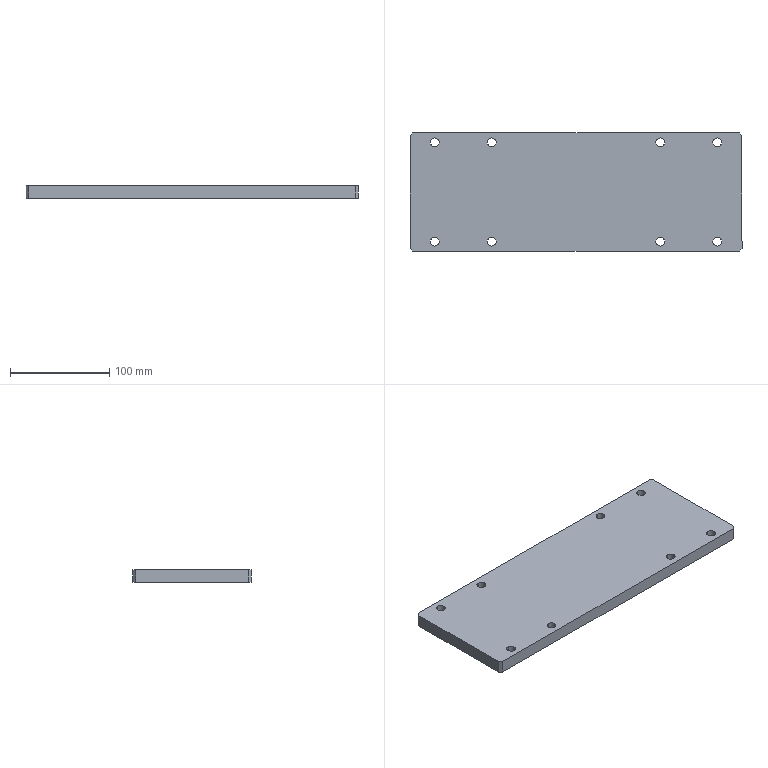Component | SolidWorks | STE21014.01-42-2 | 1 solid | 26 faces | box 335 x 120 x 13 mm | volume 515750 mm3 | cylinder 16 | plane 10 | commonest cylinder face diameters 9 x16 | material Q235
build123d program:
from build123d import *

# Parameters (mm, degrees)
SKETCH1_W            = 335
SKETCH1_H            = 120
BOSS_EXTRUDE1_DEPTH  = 13
M8_CLEARANCE_HOLE1_D = 9
CHAMFER1_SIZE        = 3


with BuildPart() as part:
    # Sketch1 → Boss-Extrude1 (new body)
    with BuildSketch(Plane(origin=(0, 0, 0), x_dir=(1, 0, 0), z_dir=(0, 1, 0))):
        Rectangle(SKETCH1_W, SKETCH1_H)
    extrude(amount=BOSS_EXTRUDE1_DEPTH)

    # M8 Clearance Hole1 (through all)
    with Locations(Plane(origin=(0, 13, 0), x_dir=(1, 0, 0), z_dir=(0, 1, 0))):
        with Locations((-142.5, -50), (-85, -50), (85, -50), (142.5, -50), (-142.5, 50), (-85, 50), (85, 50), (142.5, 50)):
            Hole(M8_CLEARANCE_HOLE1_D / 2)

    # Chamfer1
    chamfer1_edges = [part.edges().sort_by_distance(p)[0] for p in [
        (-167.5, 6.5, -60),
        (167.5, 6.5, -60),
        (167.5, 6.5, 60),
        (-167.5, 6.5, 60),
    ]]
    chamfer(chamfer1_edges, length=CHAMFER1_SIZE)


solid = part.part

# Placed as in the assembly
solid = solid.moved(Location((137.5, 890, -673), (90, 0, 0)))
STEP:
#1=COLOUR_RGB('',0.7922,0.8196,0.9333);
#2=FILL_AREA_STYLE_COLOUR('',#1);
#3=FILL_AREA_STYLE('',(#2));
#4=SURFACE_STYLE_FILL_AREA(#3);
#5=SURFACE_SIDE_STYLE('',(#4));
#6=SURFACE_STYLE_USAGE(.BOTH.,#5);
#7=PRESENTATION_STYLE_ASSIGNMENT((#6));
#8=CARTESIAN_POINT('',(-0.1969,36.831,-25.984));
#9=VERTEX_POINT('',#8);
#10=CARTESIAN_POINT('',(-0.1969,37.185,-25.984));
#11=VERTEX_POINT('',#10);
#12=CARTESIAN_POINT('',(-0.1969,37.008,-25.984));
#13=DIRECTION('',(0.,-0.,-1.));
#14=DIRECTION('',(-0.,1.,0.));
#15=AXIS2_PLACEMENT_3D('',#12,#13,#14);
#16=CIRCLE('',#15,0.1772);
#17=EDGE_CURVE('',#9,#11,#16,.T.);
#18=ORIENTED_EDGE('',*,*,#17,.F.);
#19=CARTESIAN_POINT('',(-0.1969,36.831,-26.496));
#20=VERTEX_POINT('',#19);
#21=CARTESIAN_POINT('',(-0.1969,36.831,-26.496));
#22=DIRECTION('',(0.,-0.,-1.));
#23=VECTOR('',#22,39.37);
#24=LINE('',#21,#23);
#25=EDGE_CURVE('',#9,#20,#24,.T.);
#26=ORIENTED_EDGE('',*,*,#25,.T.);
#27=CARTESIAN_POINT('',(-0.1969,37.185,-26.496));
#28=VERTEX_POINT('',#27);
#29=CARTESIAN_POINT('',(-0.1969,37.008,-26.496));
#30=DIRECTION('',(0.,-0.,-1.));
#31=DIRECTION('',(-0.,1.,0.));
#32=AXIS2_PLACEMENT_3D('',#29,#30,#31);
#33=CIRCLE('',#32,0.1772);
#34=EDGE_CURVE('',#20,#28,#33,.T.);
#35=ORIENTED_EDGE('',*,*,#34,.T.);
#36=CARTESIAN_POINT('',(-0.1969,37.185,-26.496));
#37=DIRECTION('',(0.,-0.,-1.));
#38=VECTOR('',#37,39.37);
#39=LINE('',#36,#38);
#40=EDGE_CURVE('',#11,#28,#39,.T.);
#41=ORIENTED_EDGE('',*,*,#40,.F.);
#42=EDGE_LOOP('',(#18,#26,#35,#41));
#43=FACE_OUTER_BOUND('',#42,.T.);
#44=CARTESIAN_POINT('',(-0.1969,37.008,-26.496));
#45=DIRECTION('',(0.,-0.,-1.));
#46=DIRECTION('',(-0.,1.,0.));
#47=AXIS2_PLACEMENT_3D('',#44,#45,#46);
#48=CYLINDRICAL_SURFACE('',#47,0.1772);
#49=ADVANCED_FACE('',(#43),#48,.F.);
#50=CARTESIAN_POINT('',(2.067,36.831,-25.984));
#51=VERTEX_POINT('',#50);
#52=CARTESIAN_POINT('',(2.067,37.185,-25.984));
#53=VERTEX_POINT('',#52);
#54=CARTESIAN_POINT('',(2.067,37.008,-25.984));
#55=DIRECTION('',(0.,-0.,-1.));
#56=DIRECTION('',(-0.,1.,0.));
#57=AXIS2_PLACEMENT_3D('',#54,#55,#56);
#58=CIRCLE('',#57,0.1772);
#59=EDGE_CURVE('',#51,#53,#58,.T.);
#60=ORIENTED_EDGE('',*,*,#59,.F.);
#61=CARTESIAN_POINT('',(2.067,36.831,-26.496));
#62=VERTEX_POINT('',#61);
#63=CARTESIAN_POINT('',(2.067,36.831,-26.496));
#64=DIRECTION('',(0.,-0.,-1.));
#65=VECTOR('',#64,39.37);
#66=LINE('',#63,#65);
#67=EDGE_CURVE('',#51,#62,#66,.T.);
#68=ORIENTED_EDGE('',*,*,#67,.T.);
#69=CARTESIAN_POINT('',(2.067,37.185,-26.496));
#70=VERTEX_POINT('',#69);
#71=CARTESIAN_POINT('',(2.067,37.008,-26.496));
#72=DIRECTION('',(0.,-0.,-1.));
#73=DIRECTION('',(-0.,1.,0.));
#74=AXIS2_PLACEMENT_3D('',#71,#72,#73);
#75=CIRCLE('',#74,0.1772);
#76=EDGE_CURVE('',#62,#70,#75,.T.);
#77=ORIENTED_EDGE('',*,*,#76,.T.);
#78=CARTESIAN_POINT('',(2.067,37.185,-26.496));
#79=DIRECTION('',(0.,-0.,-1.));
#80=VECTOR('',#79,39.37);
#81=LINE('',#78,#80);
#82=EDGE_CURVE('',#53,#70,#81,.T.);
#83=ORIENTED_EDGE('',*,*,#82,.F.);
#84=EDGE_LOOP('',(#60,#68,#77,#83));
#85=FACE_OUTER_BOUND('',#84,.T.);
#86=CARTESIAN_POINT('',(2.067,37.008,-26.496));
#87=DIRECTION('',(0.,-0.,-1.));
#88=DIRECTION('',(-0.,1.,0.));
#89=AXIS2_PLACEMENT_3D('',#86,#87,#88);
#90=CYLINDRICAL_SURFACE('',#89,0.1772);
#91=ADVANCED_FACE('',(#85),#90,.F.);
#92=CARTESIAN_POINT('',(8.76,36.831,-25.984));
#93=VERTEX_POINT('',#92);
#94=CARTESIAN_POINT('',(8.76,37.185,-25.984));
#95=VERTEX_POINT('',#94);
#96=CARTESIAN_POINT('',(8.76,37.008,-25.984));
#97=DIRECTION('',(0.,-0.,-1.));
#98=DIRECTION('',(-0.,1.,0.));
#99=AXIS2_PLACEMENT_3D('',#96,#97,#98);
#100=CIRCLE('',#99,0.1772);
#101=EDGE_CURVE('',#93,#95,#100,.T.);
#102=ORIENTED_EDGE('',*,*,#101,.F.);
#103=CARTESIAN_POINT('',(8.76,36.831,-26.496));
#104=VERTEX_POINT('',#103);
#105=CARTESIAN_POINT('',(8.76,36.831,-26.496));
#106=DIRECTION('',(0.,-0.,-1.));
#107=VECTOR('',#106,39.37);
#108=LINE('',#105,#107);
#109=EDGE_CURVE('',#93,#104,#108,.T.);
#110=ORIENTED_EDGE('',*,*,#109,.T.);
#111=CARTESIAN_POINT('',(8.76,37.185,-26.496));
#112=VERTEX_POINT('',#111);
#113=CARTESIAN_POINT('',(8.76,37.008,-26.496));
#114=DIRECTION('',(0.,-0.,-1.));
#115=DIRECTION('',(-0.,1.,0.));
#116=AXIS2_PLACEMENT_3D('',#113,#114,#115);
#117=CIRCLE('',#116,0.1772);
#118=EDGE_CURVE('',#104,#112,#117,.T.);
#119=ORIENTED_EDGE('',*,*,#118,.T.);
#120=CARTESIAN_POINT('',(8.76,37.185,-26.496));
#121=DIRECTION('',(0.,-0.,-1.));
#122=VECTOR('',#121,39.37);
#123=LINE('',#120,#122);
#124=EDGE_CURVE('',#95,#112,#123,.T.);
#125=ORIENTED_EDGE('',*,*,#124,.F.);
#126=EDGE_LOOP('',(#102,#110,#119,#125));
#127=FACE_OUTER_BOUND('',#126,.T.);
#128=CARTESIAN_POINT('',(8.76,37.008,-26.496));
#129=DIRECTION('',(0.,-0.,-1.));
#130=DIRECTION('',(-0.,1.,0.));
#131=AXIS2_PLACEMENT_3D('',#128,#129,#130);
#132=CYLINDRICAL_SURFACE('',#131,0.1772);
#133=ADVANCED_FACE('',(#127),#132,.F.);
#134=CARTESIAN_POINT('',(11.024,36.831,-25.984));
#135=VERTEX_POINT('',#134);
#136=CARTESIAN_POINT('',(11.024,37.185,-25.984));
#137=VERTEX_POINT('',#136);
#138=CARTESIAN_POINT('',(11.024,37.008,-25.984));
#139=DIRECTION('',(0.,-0.,-1.));
#140=DIRECTION('',(0.,1.,0.));
#141=AXIS2_PLACEMENT_3D('',#138,#139,#140);
#142=CIRCLE('',#141,0.1772);
#143=EDGE_CURVE('',#135,#137,#142,.T.);
#144=ORIENTED_EDGE('',*,*,#143,.F.);
#145=CARTESIAN_POINT('',(11.024,36.831,-26.496));
#146=VERTEX_POINT('',#145);
#147=CARTESIAN_POINT('',(11.024,36.831,-26.496));
#148=DIRECTION('',(0.,-0.,-1.));
#149=VECTOR('',#148,39.37);
#150=LINE('',#147,#149);
#151=EDGE_CURVE('',#135,#146,#150,.T.);
#152=ORIENTED_EDGE('',*,*,#151,.T.);
#153=CARTESIAN_POINT('',(11.024,37.185,-26.496));
#154=VERTEX_POINT('',#153);
#155=CARTESIAN_POINT('',(11.024,37.008,-26.496));
#156=DIRECTION('',(0.,-0.,-1.));
#157=DIRECTION('',(0.,1.,0.));
#158=AXIS2_PLACEMENT_3D('',#155,#156,#157);
#159=CIRCLE('',#158,0.1772);
#160=EDGE_CURVE('',#146,#154,#159,.T.);
#161=ORIENTED_EDGE('',*,*,#160,.T.);
#162=CARTESIAN_POINT('',(11.024,37.185,-26.496));
#163=DIRECTION('',(0.,-0.,-1.));
#164=VECTOR('',#163,39.37);
#165=LINE('',#162,#164);
#166=EDGE_CURVE('',#137,#154,#165,.T.);
#167=ORIENTED_EDGE('',*,*,#166,.F.);
#168=EDGE_LOOP('',(#144,#152,#161,#167));
#169=FACE_OUTER_BOUND('',#168,.T.);
#170=CARTESIAN_POINT('',(11.024,37.008,-26.496));
#171=DIRECTION('',(0.,-0.,-1.));
#172=DIRECTION('',(0.,1.,0.));
#173=AXIS2_PLACEMENT_3D('',#170,#171,#172);
#174=CYLINDRICAL_SURFACE('',#173,0.1772);
#175=ADVANCED_FACE('',(#169),#174,.F.);
#176=CARTESIAN_POINT('',(-0.1969,32.894,-25.984));
#177=VERTEX_POINT('',#176);
#178=CARTESIAN_POINT('',(-0.1969,33.248,-25.984));
#179=VERTEX_POINT('',#178);
#180=CARTESIAN_POINT('',(-0.1969,33.071,-25.984));
#181=DIRECTION('',(0.,-0.,-1.));
#182=DIRECTION('',(-0.,1.,0.));
#183=AXIS2_PLACEMENT_3D('',#180,#181,#182);
#184=CIRCLE('',#183,0.1772);
#185=EDGE_CURVE('',#177,#179,#184,.T.);
#186=ORIENTED_EDGE('',*,*,#185,.F.);
#187=CARTESIAN_POINT('',(-0.1969,32.894,-26.496));
#188=VERTEX_POINT('',#187);
#189=CARTESIAN_POINT('',(-0.1969,32.894,-26.496));
#190=DIRECTION('',(0.,-0.,-1.));
#191=VECTOR('',#190,39.37);
#192=LINE('',#189,#191);
#193=EDGE_CURVE('',#177,#188,#192,.T.);
#194=ORIENTED_EDGE('',*,*,#193,.T.);
#195=CARTESIAN_POINT('',(-0.1969,33.248,-26.496));
#196=VERTEX_POINT('',#195);
#197=CARTESIAN_POINT('',(-0.1969,33.071,-26.496));
#198=DIRECTION('',(0.,-0.,-1.));
#199=DIRECTION('',(-0.,1.,0.));
#200=AXIS2_PLACEMENT_3D('',#197,#198,#199);
#201=CIRCLE('',#200,0.1772);
#202=EDGE_CURVE('',#188,#196,#201,.T.);
#203=ORIENTED_EDGE('',*,*,#202,.T.);
#204=CARTESIAN_POINT('',(-0.1969,33.248,-26.496));
#205=DIRECTION('',(0.,-0.,-1.));
#206=VECTOR('',#205,39.37);
#207=LINE('',#204,#206);
#208=EDGE_CURVE('',#179,#196,#207,.T.);
#209=ORIENTED_EDGE('',*,*,#208,.F.);
#210=EDGE_LOOP('',(#186,#194,#203,#209));
#211=FACE_OUTER_BOUND('',#210,.T.);
#212=CARTESIAN_POINT('',(-0.1969,33.071,-26.496));
#213=DIRECTION('',(0.,-0.,-1.));
#214=DIRECTION('',(-0.,1.,0.));
#215=AXIS2_PLACEMENT_3D('',#212,#213,#214);
#216=CYLINDRICAL_SURFACE('',#215,0.1772);
#217=ADVANCED_FACE('',(#211),#216,.F.);
#218=CARTESIAN_POINT('',(2.067,32.894,-25.984));
#219=VERTEX_POINT('',#218);
#220=CARTESIAN_POINT('',(2.067,33.248,-25.984));
#221=VERTEX_POINT('',#220);
#222=CARTESIAN_POINT('',(2.067,33.071,-25.984));
#223=DIRECTION('',(0.,-0.,-1.));
#224=DIRECTION('',(-0.,1.,0.));
#225=AXIS2_PLACEMENT_3D('',#222,#223,#224);
#226=CIRCLE('',#225,0.1772);
#227=EDGE_CURVE('',#219,#221,#226,.T.);
#228=ORIENTED_EDGE('',*,*,#227,.F.);
#229=CARTESIAN_POINT('',(2.067,32.894,-26.496));
#230=VERTEX_POINT('',#229);
#231=CARTESIAN_POINT('',(2.067,32.894,-26.496));
#232=DIRECTION('',(0.,-0.,-1.));
#233=VECTOR('',#232,39.37);
#234=LINE('',#231,#233);
#235=EDGE_CURVE('',#219,#230,#234,.T.);
#236=ORIENTED_EDGE('',*,*,#235,.T.);
#237=CARTESIAN_POINT('',(2.067,33.248,-26.496));
#238=VERTEX_POINT('',#237);
#239=CARTESIAN_POINT('',(2.067,33.071,-26.496));
#240=DIRECTION('',(0.,-0.,-1.));
#241=DIRECTION('',(-0.,1.,0.));
#242=AXIS2_PLACEMENT_3D('',#239,#240,#241);
#243=CIRCLE('',#242,0.1772);
#244=EDGE_CURVE('',#230,#238,#243,.T.);
#245=ORIENTED_EDGE('',*,*,#244,.T.);
#246=CARTESIAN_POINT('',(2.067,33.248,-26.496));
#247=DIRECTION('',(0.,-0.,-1.));
#248=VECTOR('',#247,39.37);
#249=LINE('',#246,#248);
#250=EDGE_CURVE('',#221,#238,#249,.T.);
#251=ORIENTED_EDGE('',*,*,#250,.F.);
#252=EDGE_LOOP('',(#228,#236,#245,#251));
#253=FACE_OUTER_BOUND('',#252,.T.);
#254=CARTESIAN_POINT('',(2.067,33.071,-26.496));
#255=DIRECTION('',(0.,-0.,-1.));
#256=DIRECTION('',(-0.,1.,0.));
#257=AXIS2_PLACEMENT_3D('',#254,#255,#256);
#258=CYLINDRICAL_SURFACE('',#257,0.1772);
#259=ADVANCED_FACE('',(#253),#258,.F.);
#260=CARTESIAN_POINT('',(8.76,32.894,-25.984));
#261=VERTEX_POINT('',#260);
#262=CARTESIAN_POINT('',(8.76,33.248,-25.984));
#263=VERTEX_POINT('',#262);
#264=CARTESIAN_POINT('',(8.76,33.071,-25.984));
#265=DIRECTION('',(0.,-0.,-1.));
#266=DIRECTION('',(-0.,1.,0.));
#267=AXIS2_PLACEMENT_3D('',#264,#265,#266);
#268=CIRCLE('',#267,0.1772);
#269=EDGE_CURVE('',#261,#263,#268,.T.);
#270=ORIENTED_EDGE('',*,*,#269,.F.);
#271=CARTESIAN_POINT('',(8.76,32.894,-26.496));
#272=VERTEX_POINT('',#271);
#273=CARTESIAN_POINT('',(8.76,32.894,-26.496));
#274=DIRECTION('',(0.,-0.,-1.));
#275=VECTOR('',#274,39.37);
#276=LINE('',#273,#275);
#277=EDGE_CURVE('',#261,#272,#276,.T.);
#278=ORIENTED_EDGE('',*,*,#277,.T.);
#279=CARTESIAN_POINT('',(8.76,33.248,-26.496));
#280=VERTEX_POINT('',#279);
#281=CARTESIAN_POINT('',(8.76,33.071,-26.496));
#282=DIRECTION('',(0.,-0.,-1.));
#283=DIRECTION('',(-0.,1.,0.));
#284=AXIS2_PLACEMENT_3D('',#281,#282,#283);
#285=CIRCLE('',#284,0.1772);
#286=EDGE_CURVE('',#272,#280,#285,.T.);
#287=ORIENTED_EDGE('',*,*,#286,.T.);
#288=CARTESIAN_POINT('',(8.76,33.248,-26.496));
#289=DIRECTION('',(0.,-0.,-1.));
#290=VECTOR('',#289,39.37);
#291=LINE('',#288,#290);
#292=EDGE_CURVE('',#263,#280,#291,.T.);
#293=ORIENTED_EDGE('',*,*,#292,.F.);
#294=EDGE_LOOP('',(#270,#278,#287,#293));
#295=FACE_OUTER_BOUND('',#294,.T.);
#296=CARTESIAN_POINT('',(8.76,33.071,-26.496));
#297=DIRECTION('',(0.,-0.,-1.));
#298=DIRECTION('',(-0.,1.,0.));
#299=AXIS2_PLACEMENT_3D('',#296,#297,#298);
#300=CYLINDRICAL_SURFACE('',#299,0.1772);
#301=ADVANCED_FACE('',(#295),#300,.F.);
#302=CARTESIAN_POINT('',(11.024,32.894,-25.984));
#303=VERTEX_POINT('',#302);
#304=CARTESIAN_POINT('',(11.024,33.248,-25.984));
#305=VERTEX_POINT('',#304);
#306=CARTESIAN_POINT('',(11.024,33.071,-25.984));
#307=DIRECTION('',(0.,-0.,-1.));
#308=DIRECTION('',(0.,1.,0.));
#309=AXIS2_PLACEMENT_3D('',#306,#307,#308);
#310=CIRCLE('',#309,0.1772);
#311=EDGE_CURVE('',#303,#305,#310,.T.);
#312=ORIENTED_EDGE('',*,*,#311,.F.);
#313=CARTESIAN_POINT('',(11.024,32.894,-26.496));
#314=VERTEX_POINT('',#313);
#315=CARTESIAN_POINT('',(11.024,32.894,-26.496));
#316=DIRECTION('',(0.,-0.,-1.));
#317=VECTOR('',#316,39.37);
#318=LINE('',#315,#317);
#319=EDGE_CURVE('',#303,#314,#318,.T.);
#320=ORIENTED_EDGE('',*,*,#319,.T.);
#321=CARTESIAN_POINT('',(11.024,33.248,-26.496));
#322=VERTEX_POINT('',#321);
#323=CARTESIAN_POINT('',(11.024,33.071,-26.496));
#324=DIRECTION('',(0.,-0.,-1.));
#325=DIRECTION('',(0.,1.,0.));
#326=AXIS2_PLACEMENT_3D('',#323,#324,#325);
#327=CIRCLE('',#326,0.1772);
#328=EDGE_CURVE('',#314,#322,#327,.T.);
#329=ORIENTED_EDGE('',*,*,#328,.T.);
#330=CARTESIAN_POINT('',(11.024,33.248,-26.496));
#331=DIRECTION('',(0.,-0.,-1.));
#332=VECTOR('',#331,39.37);
#333=LINE('',#330,#332);
#334=EDGE_CURVE('',#305,#322,#333,.T.);
#335=ORIENTED_EDGE('',*,*,#334,.F.);
#336=EDGE_LOOP('',(#312,#320,#329,#335));
#337=FACE_OUTER_BOUND('',#336,.T.);
#338=CARTESIAN_POINT('',(11.024,33.071,-26.496));
#339=DIRECTION('',(0.,-0.,-1.));
#340=DIRECTION('',(0.,1.,0.));
#341=AXIS2_PLACEMENT_3D('',#338,#339,#340);
#342=CYLINDRICAL_SURFACE('',#341,0.1772);
#343=ADVANCED_FACE('',(#337),#342,.F.);
#344=CARTESIAN_POINT('',(-1.181,32.795,-26.496));
#345=VERTEX_POINT('',#344);
#346=CARTESIAN_POINT('',(-1.181,37.283,-26.496));
#347=VERTEX_POINT('',#346);
#348=CARTESIAN_POINT('',(-1.181,37.402,-26.496));
#349=DIRECTION('',(-0.,1.,-0.));
#350=VECTOR('',#349,39.37);
#351=LINE('',#348,#350);
#352=EDGE_CURVE('',#345,#347,#351,.T.);
#353=ORIENTED_EDGE('',*,*,#352,.F.);
#354=CARTESIAN_POINT('',(-1.181,32.795,-25.984));
#355=VERTEX_POINT('',#354);
#356=CARTESIAN_POINT('',(-1.181,32.795,-26.496));
#357=DIRECTION('',(-0.,0.,1.));
#358=VECTOR('',#357,39.37);
#359=LINE('',#356,#358);
#360=EDGE_CURVE('',#345,#355,#359,.T.);
#361=ORIENTED_EDGE('',*,*,#360,.T.);
#362=CARTESIAN_POINT('',(-1.181,37.283,-25.984));
#363=VERTEX_POINT('',#362);
#364=CARTESIAN_POINT('',(-1.181,37.402,-25.984));
#365=DIRECTION('',(-0.,1.,-0.));
#366=VECTOR('',#365,39.37);
#367=LINE('',#364,#366);
#368=EDGE_CURVE('',#355,#363,#367,.T.);
#369=ORIENTED_EDGE('',*,*,#368,.T.);
#370=CARTESIAN_POINT('',(-1.181,37.283,-26.496));
#371=DIRECTION('',(0.,-0.,-1.));
#372=VECTOR('',#371,39.37);
#373=LINE('',#370,#372);
#374=EDGE_CURVE('',#363,#347,#373,.T.);
#375=ORIENTED_EDGE('',*,*,#374,.T.);
#376=EDGE_LOOP('',(#353,#361,#369,#375));
#377=FACE_OUTER_BOUND('',#376,.T.);
#378=CARTESIAN_POINT('',(-1.181,37.402,-26.496));
#379=DIRECTION('',(1.,0.,0.));
#380=DIRECTION('',(0.,-1.,0.));
#381=AXIS2_PLACEMENT_3D('',#378,#379,#380);
#382=PLANE('',#381);
#383=ADVANCED_FACE('',(#377),#382,.F.);
#384=CARTESIAN_POINT('',(-1.063,37.402,-25.984));
#385=VERTEX_POINT('',#384);
#386=CARTESIAN_POINT('',(11.89,37.402,-25.984));
#387=VERTEX_POINT('',#386);
#388=CARTESIAN_POINT('',(12.008,37.402,-25.984));
#389=DIRECTION('',(1.,0.,0.));
#390=VECTOR('',#389,39.37);
#391=LINE('',#388,#390);
#392=EDGE_CURVE('',#385,#387,#391,.T.);
#393=ORIENTED_EDGE('',*,*,#392,.T.);
#394=CARTESIAN_POINT('',(11.89,37.402,-26.496));
#395=VERTEX_POINT('',#394);
#396=CARTESIAN_POINT('',(11.89,37.402,-26.496));
#397=DIRECTION('',(0.,-0.,-1.));
#398=VECTOR('',#397,39.37);
#399=LINE('',#396,#398);
#400=EDGE_CURVE('',#387,#395,#399,.T.);
#401=ORIENTED_EDGE('',*,*,#400,.T.);
#402=CARTESIAN_POINT('',(-1.063,37.402,-26.496));
#403=VERTEX_POINT('',#402);
#404=CARTESIAN_POINT('',(12.008,37.402,-26.496));
#405=DIRECTION('',(1.,0.,0.));
#406=VECTOR('',#405,39.37);
#407=LINE('',#404,#406);
#408=EDGE_CURVE('',#403,#395,#407,.T.);
#409=ORIENTED_EDGE('',*,*,#408,.F.);
#410=CARTESIAN_POINT('',(-1.063,37.402,-26.496));
#411=DIRECTION('',(-0.,0.,1.));
#412=VECTOR('',#411,39.37);
#413=LINE('',#410,#412);
#414=EDGE_CURVE('',#403,#385,#413,.T.);
#415=ORIENTED_EDGE('',*,*,#414,.T.);
#416=EDGE_LOOP('',(#393,#401,#409,#415));
#417=FACE_OUTER_BOUND('',#416,.T.);
#418=CARTESIAN_POINT('',(12.008,37.402,-26.496));
#419=DIRECTION('',(0.,-1.,0.));
#420=DIRECTION('',(-1.,-0.,-0.));
#421=AXIS2_PLACEMENT_3D('',#418,#419,#420);
#422=PLANE('',#421);
#423=ADVANCED_FACE('',(#417),#422,.F.);
#424=CARTESIAN_POINT('',(12.008,37.283,-26.496));
#425=VERTEX_POINT('',#424);
#426=CARTESIAN_POINT('',(12.008,32.795,-26.496));
#427=VERTEX_POINT('',#426);
#428=CARTESIAN_POINT('',(12.008,37.402,-26.496));
#429=DIRECTION('',(0.,-1.,0.));
#430=VECTOR('',#429,39.37);
#431=LINE('',#428,#430);
#432=EDGE_CURVE('',#425,#427,#431,.T.);
#433=ORIENTED_EDGE('',*,*,#432,.F.);
#434=CARTESIAN_POINT('',(12.008,37.283,-25.984));
#435=VERTEX_POINT('',#434);
#436=CARTESIAN_POINT('',(12.008,37.283,-26.496));
#437=DIRECTION('',(-0.,0.,1.));
#438=VECTOR('',#437,39.37);
#439=LINE('',#436,#438);
#440=EDGE_CURVE('',#425,#435,#439,.T.);
#441=ORIENTED_EDGE('',*,*,#440,.T.);
#442=CARTESIAN_POINT('',(12.008,32.795,-25.984));
#443=VERTEX_POINT('',#442);
#444=CARTESIAN_POINT('',(12.008,37.402,-25.984));
#445=DIRECTION('',(0.,-1.,0.));
#446=VECTOR('',#445,39.37);
#447=LINE('',#444,#446);
#448=EDGE_CURVE('',#435,#443,#447,.T.);
#449=ORIENTED_EDGE('',*,*,#448,.T.);
#450=CARTESIAN_POINT('',(12.008,32.795,-26.496));
#451=DIRECTION('',(0.,-0.,-1.));
#452=VECTOR('',#451,39.37);
#453=LINE('',#450,#452);
#454=EDGE_CURVE('',#443,#427,#453,.T.);
#455=ORIENTED_EDGE('',*,*,#454,.T.);
#456=EDGE_LOOP('',(#433,#441,#449,#455));
#457=FACE_OUTER_BOUND('',#456,.T.);
#458=CARTESIAN_POINT('',(12.008,37.402,-26.496));
#459=DIRECTION('',(-1.,-0.,-0.));
#460=DIRECTION('',(-0.,1.,-0.));
#461=AXIS2_PLACEMENT_3D('',#458,#459,#460);
#462=PLANE('',#461);
#463=ADVANCED_FACE('',(#457),#462,.F.);
#464=CARTESIAN_POINT('',(11.89,32.677,-26.496));
#465=VERTEX_POINT('',#464);
#466=CARTESIAN_POINT('',(-1.063,32.677,-26.496));
#467=VERTEX_POINT('',#466);
#468=CARTESIAN_POINT('',(12.008,32.677,-26.496));
#469=DIRECTION('',(-1.,-0.,-0.));
#470=VECTOR('',#469,39.37);
#471=LINE('',#468,#470);
#472=EDGE_CURVE('',#465,#467,#471,.T.);
#473=ORIENTED_EDGE('',*,*,#472,.F.);
#474=CARTESIAN_POINT('',(11.89,32.677,-25.984));
#475=VERTEX_POINT('',#474);
#476=CARTESIAN_POINT('',(11.89,32.677,-26.496));
#477=DIRECTION('',(-0.,0.,1.));
#478=VECTOR('',#477,39.37);
#479=LINE('',#476,#478);
#480=EDGE_CURVE('',#465,#475,#479,.T.);
#481=ORIENTED_EDGE('',*,*,#480,.T.);
#482=CARTESIAN_POINT('',(-1.063,32.677,-25.984));
#483=VERTEX_POINT('',#482);
#484=CARTESIAN_POINT('',(12.008,32.677,-25.984));
#485=DIRECTION('',(-1.,-0.,-0.));
#486=VECTOR('',#485,39.37);
#487=LINE('',#484,#486);
#488=EDGE_CURVE('',#475,#483,#487,.T.);
#489=ORIENTED_EDGE('',*,*,#488,.T.);
#490=CARTESIAN_POINT('',(-1.063,32.677,-26.496));
#491=DIRECTION('',(0.,-0.,-1.));
#492=VECTOR('',#491,39.37);
#493=LINE('',#490,#492);
#494=EDGE_CURVE('',#483,#467,#493,.T.);
#495=ORIENTED_EDGE('',*,*,#494,.T.);
#496=EDGE_LOOP('',(#473,#481,#489,#495));
#497=FACE_OUTER_BOUND('',#496,.T.);
#498=CARTESIAN_POINT('',(12.008,32.677,-26.496));
#499=DIRECTION('',(-0.,1.,-0.));
#500=DIRECTION('',(1.,0.,0.));
#501=AXIS2_PLACEMENT_3D('',#498,#499,#500);
#502=PLANE('',#501);
#503=ADVANCED_FACE('',(#497),#502,.F.);
#504=CARTESIAN_POINT('',(-0.1969,37.008,-26.496));
#505=DIRECTION('',(0.,-0.,-1.));
#506=DIRECTION('',(-0.,1.,0.));
#507=AXIS2_PLACEMENT_3D('',#504,#505,#506);
#508=CIRCLE('',#507,0.1772);
#509=EDGE_CURVE('',#28,#20,#508,.T.);
#510=ORIENTED_EDGE('',*,*,#509,.F.);
#511=ORIENTED_EDGE('',*,*,#34,.F.);
#512=EDGE_LOOP('',(#510,#511));
#513=FACE_BOUND('',#512,.T.);
#514=CARTESIAN_POINT('',(2.067,37.008,-26.496));
#515=DIRECTION('',(0.,-0.,-1.));
#516=DIRECTION('',(-0.,1.,0.));
#517=AXIS2_PLACEMENT_3D('',#514,#515,#516);
#518=CIRCLE('',#517,0.1772);
#519=EDGE_CURVE('',#70,#62,#518,.T.);
#520=ORIENTED_EDGE('',*,*,#519,.F.);
#521=ORIENTED_EDGE('',*,*,#76,.F.);
#522=EDGE_LOOP('',(#520,#521));
#523=FACE_BOUND('',#522,.T.);
#524=CARTESIAN_POINT('',(8.76,37.008,-26.496));
#525=DIRECTION('',(0.,-0.,-1.));
#526=DIRECTION('',(-0.,1.,0.));
#527=AXIS2_PLACEMENT_3D('',#524,#525,#526);
#528=CIRCLE('',#527,0.1772);
#529=EDGE_CURVE('',#112,#104,#528,.T.);
#530=ORIENTED_EDGE('',*,*,#529,.F.);
#531=ORIENTED_EDGE('',*,*,#118,.F.);
#532=EDGE_LOOP('',(#530,#531));
#533=FACE_BOUND('',#532,.T.);
#534=CARTESIAN_POINT('',(11.024,37.008,-26.496));
#535=DIRECTION('',(0.,-0.,-1.));
#536=DIRECTION('',(0.,1.,0.));
#537=AXIS2_PLACEMENT_3D('',#534,#535,#536);
#538=CIRCLE('',#537,0.1772);
#539=EDGE_CURVE('',#154,#146,#538,.T.);
#540=ORIENTED_EDGE('',*,*,#539,.F.);
#541=ORIENTED_EDGE('',*,*,#160,.F.);
#542=EDGE_LOOP('',(#540,#541));
#543=FACE_BOUND('',#542,.T.);
#544=CARTESIAN_POINT('',(-0.1969,33.071,-26.496));
#545=DIRECTION('',(0.,-0.,-1.));
#546=DIRECTION('',(-0.,1.,0.));
#547=AXIS2_PLACEMENT_3D('',#544,#545,#546);
#548=CIRCLE('',#547,0.1772);
#549=EDGE_CURVE('',#196,#188,#548,.T.);
#550=ORIENTED_EDGE('',*,*,#549,.F.);
#551=ORIENTED_EDGE('',*,*,#202,.F.);
#552=EDGE_LOOP('',(#550,#551));
#553=FACE_BOUND('',#552,.T.);
#554=CARTESIAN_POINT('',(2.067,33.071,-26.496));
#555=DIRECTION('',(0.,-0.,-1.));
#556=DIRECTION('',(-0.,1.,0.));
#557=AXIS2_PLACEMENT_3D('',#554,#555,#556);
#558=CIRCLE('',#557,0.1772);
#559=EDGE_CURVE('',#238,#230,#558,.T.);
#560=ORIENTED_EDGE('',*,*,#559,.F.);
#561=ORIENTED_EDGE('',*,*,#244,.F.);
#562=EDGE_LOOP('',(#560,#561));
#563=FACE_BOUND('',#562,.T.);
#564=CARTESIAN_POINT('',(8.76,33.071,-26.496));
#565=DIRECTION('',(0.,-0.,-1.));
#566=DIRECTION('',(-0.,1.,0.));
#567=AXIS2_PLACEMENT_3D('',#564,#565,#566);
#568=CIRCLE('',#567,0.1772);
#569=EDGE_CURVE('',#280,#272,#568,.T.);
#570=ORIENTED_EDGE('',*,*,#569,.F.);
#571=ORIENTED_EDGE('',*,*,#286,.F.);
#572=EDGE_LOOP('',(#570,#571));
#573=FACE_BOUND('',#572,.T.);
#574=CARTESIAN_POINT('',(11.024,33.071,-26.496));
#575=DIRECTION('',(0.,-0.,-1.));
#576=DIRECTION('',(0.,1.,0.));
#577=AXIS2_PLACEMENT_3D('',#574,#575,#576);
#578=CIRCLE('',#577,0.1772);
#579=EDGE_CURVE('',#322,#314,#578,.T.);
#580=ORIENTED_EDGE('',*,*,#579,.F.);
#581=ORIENTED_EDGE('',*,*,#328,.F.);
#582=EDGE_LOOP('',(#580,#581));
#583=FACE_BOUND('',#582,.T.);
#584=ORIENTED_EDGE('',*,*,#408,.T.);
#585=CARTESIAN_POINT('',(9.833,39.459,-26.496));
#586=DIRECTION('',(0.7071,-0.7071,0.));
#587=VECTOR('',#586,39.37);
#588=LINE('',#585,#587);
#589=EDGE_CURVE('',#395,#425,#588,.T.);
#590=ORIENTED_EDGE('',*,*,#589,.T.);
#591=ORIENTED_EDGE('',*,*,#432,.T.);
#592=CARTESIAN_POINT('',(9.833,30.62,-26.496));
#593=DIRECTION('',(-0.7071,-0.7071,0.));
#594=VECTOR('',#593,39.37);
#595=LINE('',#592,#594);
#596=EDGE_CURVE('',#427,#465,#595,.T.);
#597=ORIENTED_EDGE('',*,*,#596,.T.);
#598=ORIENTED_EDGE('',*,*,#472,.T.);
#599=CARTESIAN_POINT('',(0.9941,30.62,-26.496));
#600=DIRECTION('',(-0.7071,0.7071,-0.));
#601=VECTOR('',#600,39.37);
#602=LINE('',#599,#601);
#603=EDGE_CURVE('',#467,#345,#602,.T.);
#604=ORIENTED_EDGE('',*,*,#603,.T.);
#605=ORIENTED_EDGE('',*,*,#352,.T.);
#606=CARTESIAN_POINT('',(0.9941,39.459,-26.496));
#607=DIRECTION('',(0.7071,0.7071,-0.));
#608=VECTOR('',#607,39.37);
#609=LINE('',#606,#608);
#610=EDGE_CURVE('',#347,#403,#609,.T.);
#611=ORIENTED_EDGE('',*,*,#610,.T.);
#612=EDGE_LOOP('',(#584,#590,#591,#597,#598,#604,#605,#611));
#613=FACE_OUTER_BOUND('',#612,.T.);
#614=CARTESIAN_POINT('',(5.413,35.039,-26.496));
#615=DIRECTION('',(0.,-0.,-1.));
#616=DIRECTION('',(-0.,1.,-0.));
#617=AXIS2_PLACEMENT_3D('',#614,#615,#616);
#618=PLANE('',#617);
#619=ADVANCED_FACE('',(#513,#523,#533,#543,#553,#563,#573,#583,#613),#618,.T.);
#620=CARTESIAN_POINT('',(-0.1969,37.008,-25.984));
#621=DIRECTION('',(0.,-0.,-1.));
#622=DIRECTION('',(-0.,1.,0.));
#623=AXIS2_PLACEMENT_3D('',#620,#621,#622);
#624=CIRCLE('',#623,0.1772);
#625=EDGE_CURVE('',#11,#9,#624,.T.);
#626=ORIENTED_EDGE('',*,*,#625,.T.);
#627=ORIENTED_EDGE('',*,*,#17,.T.);
#628=EDGE_LOOP('',(#626,#627));
#629=FACE_BOUND('',#628,.T.);
#630=CARTESIAN_POINT('',(2.067,37.008,-25.984));
#631=DIRECTION('',(0.,-0.,-1.));
#632=DIRECTION('',(-0.,1.,0.));
#633=AXIS2_PLACEMENT_3D('',#630,#631,#632);
#634=CIRCLE('',#633,0.1772);
#635=EDGE_CURVE('',#53,#51,#634,.T.);
#636=ORIENTED_EDGE('',*,*,#635,.T.);
#637=ORIENTED_EDGE('',*,*,#59,.T.);
#638=EDGE_LOOP('',(#636,#637));
#639=FACE_BOUND('',#638,.T.);
#640=CARTESIAN_POINT('',(8.76,37.008,-25.984));
#641=DIRECTION('',(0.,-0.,-1.));
#642=DIRECTION('',(-0.,1.,0.));
#643=AXIS2_PLACEMENT_3D('',#640,#641,#642);
#644=CIRCLE('',#643,0.1772);
#645=EDGE_CURVE('',#95,#93,#644,.T.);
#646=ORIENTED_EDGE('',*,*,#645,.T.);
#647=ORIENTED_EDGE('',*,*,#101,.T.);
#648=EDGE_LOOP('',(#646,#647));
#649=FACE_BOUND('',#648,.T.);
#650=CARTESIAN_POINT('',(11.024,37.008,-25.984));
#651=DIRECTION('',(0.,-0.,-1.));
#652=DIRECTION('',(0.,1.,0.));
#653=AXIS2_PLACEMENT_3D('',#650,#651,#652);
#654=CIRCLE('',#653,0.1772);
#655=EDGE_CURVE('',#137,#135,#654,.T.);
#656=ORIENTED_EDGE('',*,*,#655,.T.);
#657=ORIENTED_EDGE('',*,*,#143,.T.);
#658=EDGE_LOOP('',(#656,#657));
#659=FACE_BOUND('',#658,.T.);
#660=CARTESIAN_POINT('',(-0.1969,33.071,-25.984));
#661=DIRECTION('',(0.,-0.,-1.));
#662=DIRECTION('',(-0.,1.,0.));
#663=AXIS2_PLACEMENT_3D('',#660,#661,#662);
#664=CIRCLE('',#663,0.1772);
#665=EDGE_CURVE('',#179,#177,#664,.T.);
#666=ORIENTED_EDGE('',*,*,#665,.T.);
#667=ORIENTED_EDGE('',*,*,#185,.T.);
#668=EDGE_LOOP('',(#666,#667));
#669=FACE_BOUND('',#668,.T.);
#670=CARTESIAN_POINT('',(2.067,33.071,-25.984));
#671=DIRECTION('',(0.,-0.,-1.));
#672=DIRECTION('',(-0.,1.,0.));
#673=AXIS2_PLACEMENT_3D('',#670,#671,#672);
#674=CIRCLE('',#673,0.1772);
#675=EDGE_CURVE('',#221,#219,#674,.T.);
#676=ORIENTED_EDGE('',*,*,#675,.T.);
#677=ORIENTED_EDGE('',*,*,#227,.T.);
#678=EDGE_LOOP('',(#676,#677));
#679=FACE_BOUND('',#678,.T.);
#680=CARTESIAN_POINT('',(8.76,33.071,-25.984));
#681=DIRECTION('',(0.,-0.,-1.));
#682=DIRECTION('',(-0.,1.,0.));
#683=AXIS2_PLACEMENT_3D('',#680,#681,#682);
#684=CIRCLE('',#683,0.1772);
#685=EDGE_CURVE('',#263,#261,#684,.T.);
#686=ORIENTED_EDGE('',*,*,#685,.T.);
#687=ORIENTED_EDGE('',*,*,#269,.T.);
#688=EDGE_LOOP('',(#686,#687));
#689=FACE_BOUND('',#688,.T.);
#690=CARTESIAN_POINT('',(11.024,33.071,-25.984));
#691=DIRECTION('',(0.,-0.,-1.));
#692=DIRECTION('',(0.,1.,0.));
#693=AXIS2_PLACEMENT_3D('',#690,#691,#692);
#694=CIRCLE('',#693,0.1772);
#695=EDGE_CURVE('',#305,#303,#694,.T.);
#696=ORIENTED_EDGE('',*,*,#695,.T.);
#697=ORIENTED_EDGE('',*,*,#311,.T.);
#698=EDGE_LOOP('',(#696,#697));
#699=FACE_BOUND('',#698,.T.);
#700=ORIENTED_EDGE('',*,*,#448,.F.);
#701=CARTESIAN_POINT('',(12.008,37.283,-25.984));
#702=DIRECTION('',(-0.7071,0.7071,-0.));
#703=VECTOR('',#702,39.37);
#704=LINE('',#701,#703);
#705=EDGE_CURVE('',#435,#387,#704,.T.);
#706=ORIENTED_EDGE('',*,*,#705,.T.);
#707=ORIENTED_EDGE('',*,*,#392,.F.);
#708=CARTESIAN_POINT('',(-1.063,37.402,-25.984));
#709=DIRECTION('',(-0.7071,-0.7071,0.));
#710=VECTOR('',#709,39.37);
#711=LINE('',#708,#710);
#712=EDGE_CURVE('',#385,#363,#711,.T.);
#713=ORIENTED_EDGE('',*,*,#712,.T.);
#714=ORIENTED_EDGE('',*,*,#368,.F.);
#715=CARTESIAN_POINT('',(-1.181,32.795,-25.984));
#716=DIRECTION('',(0.7071,-0.7071,0.));
#717=VECTOR('',#716,39.37);
#718=LINE('',#715,#717);
#719=EDGE_CURVE('',#355,#483,#718,.T.);
#720=ORIENTED_EDGE('',*,*,#719,.T.);
#721=ORIENTED_EDGE('',*,*,#488,.F.);
#722=CARTESIAN_POINT('',(11.89,32.677,-25.984));
#723=DIRECTION('',(0.7071,0.7071,-0.));
#724=VECTOR('',#723,39.37);
#725=LINE('',#722,#724);
#726=EDGE_CURVE('',#475,#443,#725,.T.);
#727=ORIENTED_EDGE('',*,*,#726,.T.);
#728=EDGE_LOOP('',(#700,#706,#707,#713,#714,#720,#721,#727));
#729=FACE_OUTER_BOUND('',#728,.T.);
#730=CARTESIAN_POINT('',(5.413,35.039,-25.984));
#731=DIRECTION('',(0.,-0.,-1.));
#732=DIRECTION('',(-0.,1.,-0.));
#733=AXIS2_PLACEMENT_3D('',#730,#731,#732);
#734=PLANE('',#733);
#735=ADVANCED_FACE('',(#629,#639,#649,#659,#669,#679,#689,#699,#729),#734,.F.);
#736=ORIENTED_EDGE('',*,*,#319,.F.);
#737=ORIENTED_EDGE('',*,*,#695,.F.);
#738=ORIENTED_EDGE('',*,*,#334,.T.);
#739=ORIENTED_EDGE('',*,*,#579,.T.);
#740=EDGE_LOOP('',(#736,#737,#738,#739));
#741=FACE_OUTER_BOUND('',#740,.T.);
#742=CARTESIAN_POINT('',(11.024,33.071,-26.496));
#743=DIRECTION('',(0.,-0.,-1.));
#744=DIRECTION('',(0.,1.,0.));
#745=AXIS2_PLACEMENT_3D('',#742,#743,#744);
#746=CYLINDRICAL_SURFACE('',#745,0.1772);
#747=ADVANCED_FACE('',(#741),#746,.F.);
#748=ORIENTED_EDGE('',*,*,#277,.F.);
#749=ORIENTED_EDGE('',*,*,#685,.F.);
#750=ORIENTED_EDGE('',*,*,#292,.T.);
#751=ORIENTED_EDGE('',*,*,#569,.T.);
#752=EDGE_LOOP('',(#748,#749,#750,#751));
#753=FACE_OUTER_BOUND('',#752,.T.);
#754=CARTESIAN_POINT('',(8.76,33.071,-26.496));
#755=DIRECTION('',(0.,-0.,-1.));
#756=DIRECTION('',(-0.,1.,0.));
#757=AXIS2_PLACEMENT_3D('',#754,#755,#756);
#758=CYLINDRICAL_SURFACE('',#757,0.1772);
#759=ADVANCED_FACE('',(#753),#758,.F.);
#760=ORIENTED_EDGE('',*,*,#235,.F.);
#761=ORIENTED_EDGE('',*,*,#675,.F.);
#762=ORIENTED_EDGE('',*,*,#250,.T.);
#763=ORIENTED_EDGE('',*,*,#559,.T.);
#764=EDGE_LOOP('',(#760,#761,#762,#763));
#765=FACE_OUTER_BOUND('',#764,.T.);
#766=CARTESIAN_POINT('',(2.067,33.071,-26.496));
#767=DIRECTION('',(0.,-0.,-1.));
#768=DIRECTION('',(-0.,1.,0.));
#769=AXIS2_PLACEMENT_3D('',#766,#767,#768);
#770=CYLINDRICAL_SURFACE('',#769,0.1772);
#771=ADVANCED_FACE('',(#765),#770,.F.);
#772=ORIENTED_EDGE('',*,*,#193,.F.);
#773=ORIENTED_EDGE('',*,*,#665,.F.);
#774=ORIENTED_EDGE('',*,*,#208,.T.);
#775=ORIENTED_EDGE('',*,*,#549,.T.);
#776=EDGE_LOOP('',(#772,#773,#774,#775));
#777=FACE_OUTER_BOUND('',#776,.T.);
#778=CARTESIAN_POINT('',(-0.1969,33.071,-26.496));
#779=DIRECTION('',(0.,-0.,-1.));
#780=DIRECTION('',(-0.,1.,0.));
#781=AXIS2_PLACEMENT_3D('',#778,#779,#780);
#782=CYLINDRICAL_SURFACE('',#781,0.1772);
#783=ADVANCED_FACE('',(#777),#782,.F.);
#784=ORIENTED_EDGE('',*,*,#151,.F.);
#785=ORIENTED_EDGE('',*,*,#655,.F.);
#786=ORIENTED_EDGE('',*,*,#166,.T.);
#787=ORIENTED_EDGE('',*,*,#539,.T.);
#788=EDGE_LOOP('',(#784,#785,#786,#787));
#789=FACE_OUTER_BOUND('',#788,.T.);
#790=CARTESIAN_POINT('',(11.024,37.008,-26.496));
#791=DIRECTION('',(0.,-0.,-1.));
#792=DIRECTION('',(0.,1.,0.));
#793=AXIS2_PLACEMENT_3D('',#790,#791,#792);
#794=CYLINDRICAL_SURFACE('',#793,0.1772);
#795=ADVANCED_FACE('',(#789),#794,.F.);
#796=ORIENTED_EDGE('',*,*,#109,.F.);
#797=ORIENTED_EDGE('',*,*,#645,.F.);
#798=ORIENTED_EDGE('',*,*,#124,.T.);
#799=ORIENTED_EDGE('',*,*,#529,.T.);
#800=EDGE_LOOP('',(#796,#797,#798,#799));
#801=FACE_OUTER_BOUND('',#800,.T.);
#802=CARTESIAN_POINT('',(8.76,37.008,-26.496));
#803=DIRECTION('',(0.,-0.,-1.));
#804=DIRECTION('',(-0.,1.,0.));
#805=AXIS2_PLACEMENT_3D('',#802,#803,#804);
#806=CYLINDRICAL_SURFACE('',#805,0.1772);
#807=ADVANCED_FACE('',(#801),#806,.F.);
#808=ORIENTED_EDGE('',*,*,#67,.F.);
#809=ORIENTED_EDGE('',*,*,#635,.F.);
#810=ORIENTED_EDGE('',*,*,#82,.T.);
#811=ORIENTED_EDGE('',*,*,#519,.T.);
#812=EDGE_LOOP('',(#808,#809,#810,#811));
#813=FACE_OUTER_BOUND('',#812,.T.);
#814=CARTESIAN_POINT('',(2.067,37.008,-26.496));
#815=DIRECTION('',(0.,-0.,-1.));
#816=DIRECTION('',(-0.,1.,0.));
#817=AXIS2_PLACEMENT_3D('',#814,#815,#816);
#818=CYLINDRICAL_SURFACE('',#817,0.1772);
#819=ADVANCED_FACE('',(#813),#818,.F.);
#820=ORIENTED_EDGE('',*,*,#25,.F.);
#821=ORIENTED_EDGE('',*,*,#625,.F.);
#822=ORIENTED_EDGE('',*,*,#40,.T.);
#823=ORIENTED_EDGE('',*,*,#509,.T.);
#824=EDGE_LOOP('',(#820,#821,#822,#823));
#825=FACE_OUTER_BOUND('',#824,.T.);
#826=CARTESIAN_POINT('',(-0.1969,37.008,-26.496));
#827=DIRECTION('',(0.,-0.,-1.));
#828=DIRECTION('',(-0.,1.,0.));
#829=AXIS2_PLACEMENT_3D('',#826,#827,#828);
#830=CYLINDRICAL_SURFACE('',#829,0.1772);
#831=ADVANCED_FACE('',(#825),#830,.F.);
#832=ORIENTED_EDGE('',*,*,#589,.F.);
#833=ORIENTED_EDGE('',*,*,#400,.F.);
#834=ORIENTED_EDGE('',*,*,#705,.F.);
#835=ORIENTED_EDGE('',*,*,#440,.F.);
#836=EDGE_LOOP('',(#832,#833,#834,#835));
#837=FACE_OUTER_BOUND('',#836,.T.);
#838=CARTESIAN_POINT('',(12.008,37.283,-26.496));
#839=DIRECTION('',(-0.7071,-0.7071,0.));
#840=DIRECTION('',(-0.,0.,1.));
#841=AXIS2_PLACEMENT_3D('',#838,#839,#840);
#842=PLANE('',#841);
#843=ADVANCED_FACE('',(#837),#842,.F.);
#844=ORIENTED_EDGE('',*,*,#596,.F.);
#845=ORIENTED_EDGE('',*,*,#454,.F.);
#846=ORIENTED_EDGE('',*,*,#726,.F.);
#847=ORIENTED_EDGE('',*,*,#480,.F.);
#848=EDGE_LOOP('',(#844,#845,#846,#847));
#849=FACE_OUTER_BOUND('',#848,.T.);
#850=CARTESIAN_POINT('',(11.89,32.677,-26.496));
#851=DIRECTION('',(-0.7071,0.7071,-0.));
#852=DIRECTION('',(-0.,0.,1.));
#853=AXIS2_PLACEMENT_3D('',#850,#851,#852);
#854=PLANE('',#853);
#855=ADVANCED_FACE('',(#849),#854,.F.);
#856=ORIENTED_EDGE('',*,*,#603,.F.);
#857=ORIENTED_EDGE('',*,*,#494,.F.);
#858=ORIENTED_EDGE('',*,*,#719,.F.);
#859=ORIENTED_EDGE('',*,*,#360,.F.);
#860=EDGE_LOOP('',(#856,#857,#858,#859));
#861=FACE_OUTER_BOUND('',#860,.T.);
#862=CARTESIAN_POINT('',(-1.181,32.795,-26.496));
#863=DIRECTION('',(0.7071,0.7071,-0.));
#864=DIRECTION('',(-0.,0.,1.));
#865=AXIS2_PLACEMENT_3D('',#862,#863,#864);
#866=PLANE('',#865);
#867=ADVANCED_FACE('',(#861),#866,.F.);
#868=ORIENTED_EDGE('',*,*,#610,.F.);
#869=ORIENTED_EDGE('',*,*,#374,.F.);
#870=ORIENTED_EDGE('',*,*,#712,.F.);
#871=ORIENTED_EDGE('',*,*,#414,.F.);
#872=EDGE_LOOP('',(#868,#869,#870,#871));
#873=FACE_OUTER_BOUND('',#872,.T.);
#874=CARTESIAN_POINT('',(-1.063,37.402,-26.496));
#875=DIRECTION('',(0.7071,-0.7071,0.));
#876=DIRECTION('',(-0.,0.,1.));
#877=AXIS2_PLACEMENT_3D('',#874,#875,#876);
#878=PLANE('',#877);
#879=ADVANCED_FACE('',(#873),#878,.F.);
#880=CLOSED_SHELL('',(#49,#91,#133,#175,#217,#259,#301,#343,#383,#423,#463,#503,#619,#735,#747,#759,#771,#783,#795,#807,#819,#831,#843,#855,#867,#879));
#881=MANIFOLD_SOLID_BREP('',#880);
#882=STYLED_ITEM('',(#7),#881);
#883=PRESENTATION_LAYER_ASSIGNMENT('','',(#882));
#884=CARTESIAN_POINT('',(0.,0.,0.));
#885=DIRECTION('',(0.,0.,1.));
#886=DIRECTION('',(1.,0.,0.));
#887=AXIS2_PLACEMENT_3D('',#884,#885,#886);
#888=(LENGTH_UNIT()NAMED_UNIT(*)SI_UNIT($,.METRE.));
#889=LENGTH_MEASURE_WITH_UNIT(LENGTH_MEASURE(0.0254),#888);
#890=DIMENSIONAL_EXPONENTS(1.,0.,0.,0.,0.,0.,0.);
#891=(CONVERSION_BASED_UNIT('',#889)LENGTH_UNIT()NAMED_UNIT(#890));
#892=UNCERTAINTY_MEASURE_WITH_UNIT(LENGTH_MEASURE(0.00001),#891,'','');
#893=(NAMED_UNIT(*)PLANE_ANGLE_UNIT()SI_UNIT($,.RADIAN.));
#894=(NAMED_UNIT(*)SI_UNIT($,.STERADIAN.)SOLID_ANGLE_UNIT());
#895=(GEOMETRIC_REPRESENTATION_CONTEXT(3)GLOBAL_UNCERTAINTY_ASSIGNED_CONTEXT((#892))GLOBAL_UNIT_ASSIGNED_CONTEXT((#891,#893,#894))REPRESENTATION_CONTEXT('',''));
#896=ADVANCED_BREP_SHAPE_REPRESENTATION('',(#881,#887),#895);
#897=(LENGTH_UNIT()NAMED_UNIT(*)SI_UNIT($,.METRE.));
#898=LENGTH_MEASURE_WITH_UNIT(LENGTH_MEASURE(0.0254),#897);
#899=DIMENSIONAL_EXPONENTS(1.,0.,0.,0.,0.,0.,0.);
#900=(CONVERSION_BASED_UNIT('',#898)LENGTH_UNIT()NAMED_UNIT(#899));
#901=UNCERTAINTY_MEASURE_WITH_UNIT(LENGTH_MEASURE(0.00001),#900,'','');
#902=(NAMED_UNIT(*)PLANE_ANGLE_UNIT()SI_UNIT($,.RADIAN.));
#903=(NAMED_UNIT(*)SI_UNIT($,.STERADIAN.)SOLID_ANGLE_UNIT());
#904=(GEOMETRIC_REPRESENTATION_CONTEXT(3)GLOBAL_UNCERTAINTY_ASSIGNED_CONTEXT((#901))GLOBAL_UNIT_ASSIGNED_CONTEXT((#900,#902,#903))REPRESENTATION_CONTEXT('',''));
#905=MECHANICAL_DESIGN_GEOMETRIC_PRESENTATION_REPRESENTATION('',(#882),#904);